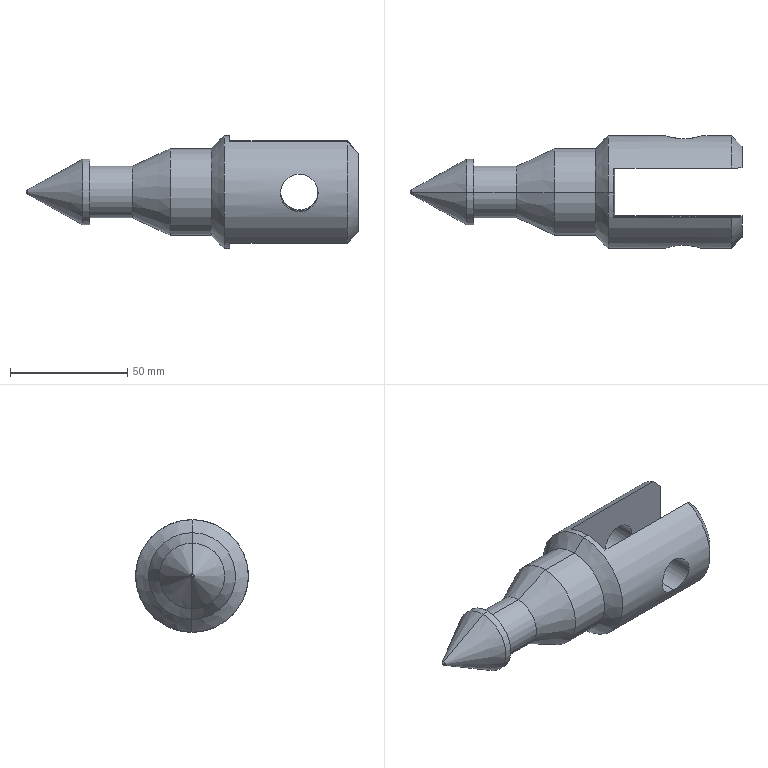Component | SolidWorks | 216InnerTubeAssembly-1_FishingSpearhead-2 | 1 solid | 37 faces | box 141.44 x 48 x 48 mm | volume 90632 mm3 | cylinder 16 | cone 14 | plane 5 | sphere 2 | commonest cylinder face diameters 16 x6 27.954 x2 22 x2 37 x2 48 x2 21 x2 | material Alloy Steel
build123d program:
from build123d import *

# Parameters (mm, degrees)
CUT_EXTRUDE3_REACH      = 147.462
CUT_EXTRUDE4_DEPTH      = 145.292
CUT_EXTRUDE4_DEPTH_BACK = 145.292
SKETCH6_R               = 8


with BuildPart() as part:
    # Model → Revolve2 (revolve)
    with BuildSketch(Plane.XY, mode=Mode.PRIVATE) as revolve2_sk:
        with BuildLine():
            Line((1.204, 10.477), (1.204, 19.473))
            Line((1.204, 19.473), (-3.3, 23.977))
            Line((-3.3, 23.977), (-55.8, 23.977))
            Line((-55.8, 23.977), (-61.3, 18.477))
            Line((-61.3, 18.477), (-78.8, 18.477))
            Line((-78.8, 18.477), (-94.884, 10.977))
            Line((-94.884, 10.977), (-114.884, 10.977))
            Line((-114.884, 10.977), (-113.165, 13.954))
            Line((-113.165, 13.954), (-116.165, 13.954))
            Line((-116.165, 13.954), (-139.725, 0.8507))
            ThreePointArc((-139.725, 0.8507), (-140.101, 0.4837), (-140.239, -0.02325))
            Line((-140.239, -0.02325), (-77.211, -0.02325))
            Line((-77.211, -0.02325), (-77.246, 7.977))
            Line((-77.246, 7.977), (-53.046, 7.977))
            Line((-53.046, 7.977), (-53.096, 10.477))
            Line((-53.096, 10.477), (1.204, 10.477))
        make_face()
    revolve(revolve2_sk.sketch.rotate(Axis((8.192, -0.02325, 0), (-1, 0, 0)), 90), axis=Axis((8.192, -0.02325, 0), (-1, 0, 0)))

    # Cut-Extrude3: up to this cone (the profile starts outside it)
    cut_extrude3_end = Plane(origin=(1.204, -0.02325, 0), z_dir=(-1, 0, 0)).offset(54.088) * Cone(0.00004956, 4652.742, 93.874, align=(Align.CENTER, Align.CENTER, Align.MIN), mode=Mode.PRIVATE)
    # Sketch5 → Cut-Extrude3 (cut, up to the surface)
    with BuildSketch(Plane(origin=(1.204, 0, 0), x_dir=(0, 0, -1), z_dir=(1, 0, 0)), mode=Mode.PRIVATE) as cut_extrude3_sk1:
        with BuildLine():
            Line((-22.614, 10.5), (22.614, 10.5))
            ThreePointArc((22.614, 10.5), (24.932, 0), (22.614, -10.5))
            Line((22.614, -10.5), (-22.614, -10.5))
            ThreePointArc((-22.614, -10.5), (-24.932, 0), (-22.614, 10.5))
        make_face()
    cut_extrude3_tool1 = extrude(cut_extrude3_sk1.sketch, amount=-CUT_EXTRUDE3_REACH, mode=Mode.PRIVATE) - cut_extrude3_end
    add(cut_extrude3_tool1.solids().sort_by_distance((1.204, 0, 0))[0], mode=Mode.SUBTRACT)

    # Sketch6 → Cut-Extrude4 (cut, two sides: drawn at the far end of the back side and taken through both)
    with BuildSketch(Plane(origin=(0, 0, 0), x_dir=(1, 0, 0), z_dir=(0, 1, 0)).offset(-CUT_EXTRUDE4_DEPTH_BACK)):
        with Locations(Location((-23.796, 0, 0), (0, 0, 354.992))):
            Circle(SKETCH6_R)
    extrude(amount=CUT_EXTRUDE4_DEPTH + CUT_EXTRUDE4_DEPTH_BACK, mode=Mode.SUBTRACT)


solid = part.part

# Placed as in the assembly
solid = solid.moved(Location((152.3, 0, 0), (1.029, 0, 0)))